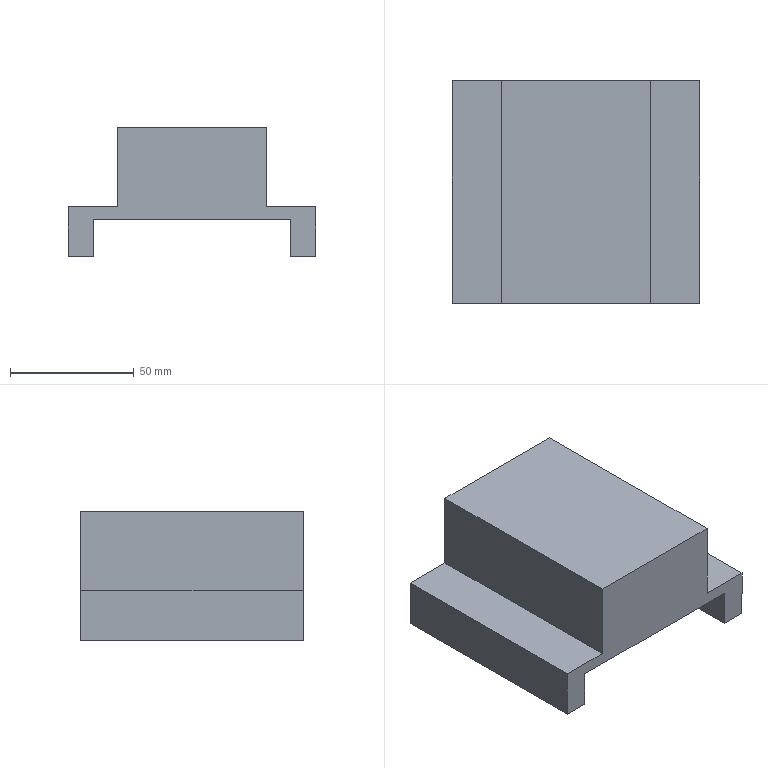Component | SolidWorks | Y-AxisAssembly-1_Y-AxisSlider-1 | 1 solid | 32 faces | box 100 x 90 x 52 mm | volume 243104 mm3 | plane 20 | cylinder 12 | commonest cylinder face diameters 6 x12
build123d program:
from build123d import *

# Parameters (mm, degrees)
BOSS_EXTRUDE1_DEPTH = 90
SKETCH2_R           = 3
CUT_EXTRUDE1_DEPTH  = 10


with BuildPart() as part:
    # Sketch1 → Boss-Extrude1 (new body)
    with BuildSketch(Plane.XY):
        Polygon((-50, 32.6), (-40, 32.6), (-40, 17.6), (40, 17.6), (40, 32.6), (50, 32.6), (50, 12.6), (30, 12.6), (30, -19.4), (-30, -19.4), (-30, 12.6), (-50, 12.6), align=None)
    extrude(amount=BOSS_EXTRUDE1_DEPTH)

    # Sketch2 → Cut-Extrude1 (cut)
    with BuildSketch(Plane(origin=(0, 32.6, 0), x_dir=(1, 0, 0), z_dir=(0, 1, 0))):
        with Locations(Location((-45, -10, 0), (0, 0, 270))):
            Circle(SKETCH2_R)
        with Locations(Location((45, -10, 0), (0, 0, 270))):
            Circle(SKETCH2_R)
        with Locations(Location((45, -45, 0), (0, 0, 270))):
            Circle(SKETCH2_R)
        with Locations(Location((45, -80, 0), (0, 0, 270))):
            Circle(SKETCH2_R)
        with Locations(Location((-45, -45, 0), (0, 0, 270))):
            Circle(SKETCH2_R)
        with Locations(Location((-45, -80, 0), (0, 0, 270))):
            Circle(SKETCH2_R)
    extrude(amount=-CUT_EXTRUDE1_DEPTH, mode=Mode.SUBTRACT)


solid = part.part

# Placed as in the assembly
solid = solid.moved(Location((-28.271, -116.882, -53.9), (-90, 0, 0)))
STEP:
#1=COLOUR_RGB('',0.7922,0.8196,0.9333);
#2=FILL_AREA_STYLE_COLOUR('',#1);
#3=FILL_AREA_STYLE('',(#2));
#4=SURFACE_STYLE_FILL_AREA(#3);
#5=SURFACE_SIDE_STYLE('',(#4));
#6=SURFACE_STYLE_USAGE(.BOTH.,#5);
#7=PRESENTATION_STYLE_ASSIGNMENT((#6));
#8=CARTESIAN_POINT('',(0.6586,-4.09,-3.012));
#9=VERTEX_POINT('',#8);
#10=CARTESIAN_POINT('',(0.6586,-4.326,-3.012));
#11=VERTEX_POINT('',#10);
#12=CARTESIAN_POINT('',(0.6586,-4.208,-3.012));
#13=DIRECTION('',(-0.,0.,-1.));
#14=DIRECTION('',(-0.,-1.,0.));
#15=AXIS2_PLACEMENT_3D('',#12,#13,#14);
#16=CIRCLE('',#15,0.1181);
#17=EDGE_CURVE('',#9,#11,#16,.T.);
#18=ORIENTED_EDGE('',*,*,#17,.F.);
#19=CARTESIAN_POINT('',(0.6586,-4.09,-3.406));
#20=VERTEX_POINT('',#19);
#21=CARTESIAN_POINT('',(0.6586,-4.09,-3.012));
#22=DIRECTION('',(-0.,0.,-1.));
#23=VECTOR('',#22,39.37);
#24=LINE('',#21,#23);
#25=EDGE_CURVE('',#9,#20,#24,.T.);
#26=ORIENTED_EDGE('',*,*,#25,.T.);
#27=CARTESIAN_POINT('',(0.6586,-4.326,-3.406));
#28=VERTEX_POINT('',#27);
#29=CARTESIAN_POINT('',(0.6586,-4.208,-3.406));
#30=DIRECTION('',(-0.,0.,-1.));
#31=DIRECTION('',(-0.,-1.,0.));
#32=AXIS2_PLACEMENT_3D('',#29,#30,#31);
#33=CIRCLE('',#32,0.1181);
#34=EDGE_CURVE('',#20,#28,#33,.T.);
#35=ORIENTED_EDGE('',*,*,#34,.T.);
#36=CARTESIAN_POINT('',(0.6586,-4.326,-3.012));
#37=DIRECTION('',(-0.,0.,-1.));
#38=VECTOR('',#37,39.37);
#39=LINE('',#36,#38);
#40=EDGE_CURVE('',#11,#28,#39,.T.);
#41=ORIENTED_EDGE('',*,*,#40,.F.);
#42=EDGE_LOOP('',(#18,#26,#35,#41));
#43=FACE_OUTER_BOUND('',#42,.T.);
#44=CARTESIAN_POINT('',(0.6586,-4.208,-3.012));
#45=DIRECTION('',(-0.,0.,-1.));
#46=DIRECTION('',(-0.,-1.,0.));
#47=AXIS2_PLACEMENT_3D('',#44,#45,#46);
#48=CYLINDRICAL_SURFACE('',#47,0.1181);
#49=ADVANCED_FACE('',(#43),#48,.F.);
#50=CARTESIAN_POINT('',(0.6586,-2.712,-3.012));
#51=VERTEX_POINT('',#50);
#52=CARTESIAN_POINT('',(0.6586,-2.948,-3.012));
#53=VERTEX_POINT('',#52);
#54=CARTESIAN_POINT('',(0.6586,-2.83,-3.012));
#55=DIRECTION('',(-0.,0.,-1.));
#56=DIRECTION('',(-0.,-1.,0.));
#57=AXIS2_PLACEMENT_3D('',#54,#55,#56);
#58=CIRCLE('',#57,0.1181);
#59=EDGE_CURVE('',#51,#53,#58,.T.);
#60=ORIENTED_EDGE('',*,*,#59,.F.);
#61=CARTESIAN_POINT('',(0.6586,-2.712,-3.406));
#62=VERTEX_POINT('',#61);
#63=CARTESIAN_POINT('',(0.6586,-2.712,-3.012));
#64=DIRECTION('',(-0.,0.,-1.));
#65=VECTOR('',#64,39.37);
#66=LINE('',#63,#65);
#67=EDGE_CURVE('',#51,#62,#66,.T.);
#68=ORIENTED_EDGE('',*,*,#67,.T.);
#69=CARTESIAN_POINT('',(0.6586,-2.948,-3.406));
#70=VERTEX_POINT('',#69);
#71=CARTESIAN_POINT('',(0.6586,-2.83,-3.406));
#72=DIRECTION('',(-0.,0.,-1.));
#73=DIRECTION('',(-0.,-1.,0.));
#74=AXIS2_PLACEMENT_3D('',#71,#72,#73);
#75=CIRCLE('',#74,0.1181);
#76=EDGE_CURVE('',#62,#70,#75,.T.);
#77=ORIENTED_EDGE('',*,*,#76,.T.);
#78=CARTESIAN_POINT('',(0.6586,-2.948,-3.012));
#79=DIRECTION('',(-0.,0.,-1.));
#80=VECTOR('',#79,39.37);
#81=LINE('',#78,#80);
#82=EDGE_CURVE('',#53,#70,#81,.T.);
#83=ORIENTED_EDGE('',*,*,#82,.F.);
#84=EDGE_LOOP('',(#60,#68,#77,#83));
#85=FACE_OUTER_BOUND('',#84,.T.);
#86=CARTESIAN_POINT('',(0.6586,-2.83,-3.012));
#87=DIRECTION('',(-0.,0.,-1.));
#88=DIRECTION('',(-0.,-1.,0.));
#89=AXIS2_PLACEMENT_3D('',#86,#87,#88);
#90=CYLINDRICAL_SURFACE('',#89,0.1181);
#91=ADVANCED_FACE('',(#85),#90,.F.);
#92=CARTESIAN_POINT('',(-2.885,-4.09,-3.012));
#93=VERTEX_POINT('',#92);
#94=CARTESIAN_POINT('',(-2.885,-4.326,-3.012));
#95=VERTEX_POINT('',#94);
#96=CARTESIAN_POINT('',(-2.885,-4.208,-3.012));
#97=DIRECTION('',(-0.,0.,-1.));
#98=DIRECTION('',(0.,-1.,0.));
#99=AXIS2_PLACEMENT_3D('',#96,#97,#98);
#100=CIRCLE('',#99,0.1181);
#101=EDGE_CURVE('',#93,#95,#100,.T.);
#102=ORIENTED_EDGE('',*,*,#101,.F.);
#103=CARTESIAN_POINT('',(-2.885,-4.09,-3.406));
#104=VERTEX_POINT('',#103);
#105=CARTESIAN_POINT('',(-2.885,-4.09,-3.012));
#106=DIRECTION('',(-0.,0.,-1.));
#107=VECTOR('',#106,39.37);
#108=LINE('',#105,#107);
#109=EDGE_CURVE('',#93,#104,#108,.T.);
#110=ORIENTED_EDGE('',*,*,#109,.T.);
#111=CARTESIAN_POINT('',(-2.885,-4.326,-3.406));
#112=VERTEX_POINT('',#111);
#113=CARTESIAN_POINT('',(-2.885,-4.208,-3.406));
#114=DIRECTION('',(-0.,0.,-1.));
#115=DIRECTION('',(0.,-1.,0.));
#116=AXIS2_PLACEMENT_3D('',#113,#114,#115);
#117=CIRCLE('',#116,0.1181);
#118=EDGE_CURVE('',#104,#112,#117,.T.);
#119=ORIENTED_EDGE('',*,*,#118,.T.);
#120=CARTESIAN_POINT('',(-2.885,-4.326,-3.012));
#121=DIRECTION('',(-0.,0.,-1.));
#122=VECTOR('',#121,39.37);
#123=LINE('',#120,#122);
#124=EDGE_CURVE('',#95,#112,#123,.T.);
#125=ORIENTED_EDGE('',*,*,#124,.F.);
#126=EDGE_LOOP('',(#102,#110,#119,#125));
#127=FACE_OUTER_BOUND('',#126,.T.);
#128=CARTESIAN_POINT('',(-2.885,-4.208,-3.012));
#129=DIRECTION('',(-0.,0.,-1.));
#130=DIRECTION('',(0.,-1.,0.));
#131=AXIS2_PLACEMENT_3D('',#128,#129,#130);
#132=CYLINDRICAL_SURFACE('',#131,0.1181);
#133=ADVANCED_FACE('',(#127),#132,.F.);
#134=CARTESIAN_POINT('',(-2.885,-2.712,-3.012));
#135=VERTEX_POINT('',#134);
#136=CARTESIAN_POINT('',(-2.885,-2.948,-3.012));
#137=VERTEX_POINT('',#136);
#138=CARTESIAN_POINT('',(-2.885,-2.83,-3.012));
#139=DIRECTION('',(-0.,0.,-1.));
#140=DIRECTION('',(0.,-1.,0.));
#141=AXIS2_PLACEMENT_3D('',#138,#139,#140);
#142=CIRCLE('',#141,0.1181);
#143=EDGE_CURVE('',#135,#137,#142,.T.);
#144=ORIENTED_EDGE('',*,*,#143,.F.);
#145=CARTESIAN_POINT('',(-2.885,-2.712,-3.406));
#146=VERTEX_POINT('',#145);
#147=CARTESIAN_POINT('',(-2.885,-2.712,-3.012));
#148=DIRECTION('',(-0.,0.,-1.));
#149=VECTOR('',#148,39.37);
#150=LINE('',#147,#149);
#151=EDGE_CURVE('',#135,#146,#150,.T.);
#152=ORIENTED_EDGE('',*,*,#151,.T.);
#153=CARTESIAN_POINT('',(-2.885,-2.948,-3.406));
#154=VERTEX_POINT('',#153);
#155=CARTESIAN_POINT('',(-2.885,-2.83,-3.406));
#156=DIRECTION('',(-0.,0.,-1.));
#157=DIRECTION('',(0.,-1.,0.));
#158=AXIS2_PLACEMENT_3D('',#155,#156,#157);
#159=CIRCLE('',#158,0.1181);
#160=EDGE_CURVE('',#146,#154,#159,.T.);
#161=ORIENTED_EDGE('',*,*,#160,.T.);
#162=CARTESIAN_POINT('',(-2.885,-2.948,-3.012));
#163=DIRECTION('',(-0.,0.,-1.));
#164=VECTOR('',#163,39.37);
#165=LINE('',#162,#164);
#166=EDGE_CURVE('',#137,#154,#165,.T.);
#167=ORIENTED_EDGE('',*,*,#166,.F.);
#168=EDGE_LOOP('',(#144,#152,#161,#167));
#169=FACE_OUTER_BOUND('',#168,.T.);
#170=CARTESIAN_POINT('',(-2.885,-2.83,-3.012));
#171=DIRECTION('',(-0.,0.,-1.));
#172=DIRECTION('',(0.,-1.,0.));
#173=AXIS2_PLACEMENT_3D('',#170,#171,#172);
#174=CYLINDRICAL_SURFACE('',#173,0.1181);
#175=ADVANCED_FACE('',(#169),#174,.F.);
#176=CARTESIAN_POINT('',(-2.885,-1.334,-3.012));
#177=VERTEX_POINT('',#176);
#178=CARTESIAN_POINT('',(-2.885,-1.57,-3.012));
#179=VERTEX_POINT('',#178);
#180=CARTESIAN_POINT('',(-2.885,-1.452,-3.012));
#181=DIRECTION('',(-0.,0.,-1.));
#182=DIRECTION('',(0.,-1.,0.));
#183=AXIS2_PLACEMENT_3D('',#180,#181,#182);
#184=CIRCLE('',#183,0.1181);
#185=EDGE_CURVE('',#177,#179,#184,.T.);
#186=ORIENTED_EDGE('',*,*,#185,.F.);
#187=CARTESIAN_POINT('',(-2.885,-1.334,-3.406));
#188=VERTEX_POINT('',#187);
#189=CARTESIAN_POINT('',(-2.885,-1.334,-3.012));
#190=DIRECTION('',(-0.,0.,-1.));
#191=VECTOR('',#190,39.37);
#192=LINE('',#189,#191);
#193=EDGE_CURVE('',#177,#188,#192,.T.);
#194=ORIENTED_EDGE('',*,*,#193,.T.);
#195=CARTESIAN_POINT('',(-2.885,-1.57,-3.406));
#196=VERTEX_POINT('',#195);
#197=CARTESIAN_POINT('',(-2.885,-1.452,-3.406));
#198=DIRECTION('',(-0.,0.,-1.));
#199=DIRECTION('',(0.,-1.,0.));
#200=AXIS2_PLACEMENT_3D('',#197,#198,#199);
#201=CIRCLE('',#200,0.1181);
#202=EDGE_CURVE('',#188,#196,#201,.T.);
#203=ORIENTED_EDGE('',*,*,#202,.T.);
#204=CARTESIAN_POINT('',(-2.885,-1.57,-3.012));
#205=DIRECTION('',(-0.,0.,-1.));
#206=VECTOR('',#205,39.37);
#207=LINE('',#204,#206);
#208=EDGE_CURVE('',#179,#196,#207,.T.);
#209=ORIENTED_EDGE('',*,*,#208,.F.);
#210=EDGE_LOOP('',(#186,#194,#203,#209));
#211=FACE_OUTER_BOUND('',#210,.T.);
#212=CARTESIAN_POINT('',(-2.885,-1.452,-3.012));
#213=DIRECTION('',(-0.,0.,-1.));
#214=DIRECTION('',(0.,-1.,0.));
#215=AXIS2_PLACEMENT_3D('',#212,#213,#214);
#216=CYLINDRICAL_SURFACE('',#215,0.1181);
#217=ADVANCED_FACE('',(#211),#216,.F.);
#218=CARTESIAN_POINT('',(0.6586,-1.334,-3.012));
#219=VERTEX_POINT('',#218);
#220=CARTESIAN_POINT('',(0.6586,-1.57,-3.012));
#221=VERTEX_POINT('',#220);
#222=CARTESIAN_POINT('',(0.6586,-1.452,-3.012));
#223=DIRECTION('',(-0.,0.,-1.));
#224=DIRECTION('',(-0.,-1.,0.));
#225=AXIS2_PLACEMENT_3D('',#222,#223,#224);
#226=CIRCLE('',#225,0.1181);
#227=EDGE_CURVE('',#219,#221,#226,.T.);
#228=ORIENTED_EDGE('',*,*,#227,.F.);
#229=CARTESIAN_POINT('',(0.6586,-1.334,-3.406));
#230=VERTEX_POINT('',#229);
#231=CARTESIAN_POINT('',(0.6586,-1.334,-3.012));
#232=DIRECTION('',(-0.,0.,-1.));
#233=VECTOR('',#232,39.37);
#234=LINE('',#231,#233);
#235=EDGE_CURVE('',#219,#230,#234,.T.);
#236=ORIENTED_EDGE('',*,*,#235,.T.);
#237=CARTESIAN_POINT('',(0.6586,-1.57,-3.406));
#238=VERTEX_POINT('',#237);
#239=CARTESIAN_POINT('',(0.6586,-1.452,-3.406));
#240=DIRECTION('',(-0.,0.,-1.));
#241=DIRECTION('',(-0.,-1.,0.));
#242=AXIS2_PLACEMENT_3D('',#239,#240,#241);
#243=CIRCLE('',#242,0.1181);
#244=EDGE_CURVE('',#230,#238,#243,.T.);
#245=ORIENTED_EDGE('',*,*,#244,.T.);
#246=CARTESIAN_POINT('',(0.6586,-1.57,-3.012));
#247=DIRECTION('',(-0.,0.,-1.));
#248=VECTOR('',#247,39.37);
#249=LINE('',#246,#248);
#250=EDGE_CURVE('',#221,#238,#249,.T.);
#251=ORIENTED_EDGE('',*,*,#250,.F.);
#252=EDGE_LOOP('',(#228,#236,#245,#251));
#253=FACE_OUTER_BOUND('',#252,.T.);
#254=CARTESIAN_POINT('',(0.6586,-1.452,-3.012));
#255=DIRECTION('',(-0.,0.,-1.));
#256=DIRECTION('',(-0.,-1.,0.));
#257=AXIS2_PLACEMENT_3D('',#254,#255,#256);
#258=CYLINDRICAL_SURFACE('',#257,0.1181);
#259=ADVANCED_FACE('',(#253),#258,.F.);
#260=CARTESIAN_POINT('',(0.8555,-1.058,-3.406));
#261=VERTEX_POINT('',#260);
#262=CARTESIAN_POINT('',(0.8555,-1.058,-2.618));
#263=VERTEX_POINT('',#262);
#264=CARTESIAN_POINT('',(0.8555,-1.058,-2.618));
#265=DIRECTION('',(0.,-0.,1.));
#266=VECTOR('',#265,39.37);
#267=LINE('',#264,#266);
#268=EDGE_CURVE('',#261,#263,#267,.T.);
#269=ORIENTED_EDGE('',*,*,#268,.T.);
#270=CARTESIAN_POINT('',(0.8555,-4.602,-2.618));
#271=VERTEX_POINT('',#270);
#272=CARTESIAN_POINT('',(0.8555,-4.602,-2.618));
#273=DIRECTION('',(0.,1.,0.));
#274=VECTOR('',#273,39.37);
#275=LINE('',#272,#274);
#276=EDGE_CURVE('',#271,#263,#275,.T.);
#277=ORIENTED_EDGE('',*,*,#276,.F.);
#278=CARTESIAN_POINT('',(0.8555,-4.602,-3.406));
#279=VERTEX_POINT('',#278);
#280=CARTESIAN_POINT('',(0.8555,-4.602,-2.618));
#281=DIRECTION('',(0.,-0.,1.));
#282=VECTOR('',#281,39.37);
#283=LINE('',#280,#282);
#284=EDGE_CURVE('',#279,#271,#283,.T.);
#285=ORIENTED_EDGE('',*,*,#284,.F.);
#286=CARTESIAN_POINT('',(0.8555,-4.602,-3.406));
#287=DIRECTION('',(0.,1.,0.));
#288=VECTOR('',#287,39.37);
#289=LINE('',#286,#288);
#290=EDGE_CURVE('',#279,#261,#289,.T.);
#291=ORIENTED_EDGE('',*,*,#290,.T.);
#292=EDGE_LOOP('',(#269,#277,#285,#291));
#293=FACE_OUTER_BOUND('',#292,.T.);
#294=CARTESIAN_POINT('',(0.8555,-4.602,-2.618));
#295=DIRECTION('',(-1.,0.,0.));
#296=DIRECTION('',(0.,1.,0.));
#297=AXIS2_PLACEMENT_3D('',#294,#295,#296);
#298=PLANE('',#297);
#299=ADVANCED_FACE('',(#293),#298,.F.);
#300=CARTESIAN_POINT('',(0.06809,-1.058,-2.618));
#301=VERTEX_POINT('',#300);
#302=CARTESIAN_POINT('',(0.06809,-1.058,-2.618));
#303=DIRECTION('',(-1.,0.,-0.));
#304=VECTOR('',#303,39.37);
#305=LINE('',#302,#304);
#306=EDGE_CURVE('',#263,#301,#305,.T.);
#307=ORIENTED_EDGE('',*,*,#306,.T.);
#308=CARTESIAN_POINT('',(0.06809,-4.602,-2.618));
#309=VERTEX_POINT('',#308);
#310=CARTESIAN_POINT('',(0.06809,-4.602,-2.618));
#311=DIRECTION('',(0.,1.,0.));
#312=VECTOR('',#311,39.37);
#313=LINE('',#310,#312);
#314=EDGE_CURVE('',#309,#301,#313,.T.);
#315=ORIENTED_EDGE('',*,*,#314,.F.);
#316=CARTESIAN_POINT('',(0.06809,-4.602,-2.618));
#317=DIRECTION('',(-1.,0.,-0.));
#318=VECTOR('',#317,39.37);
#319=LINE('',#316,#318);
#320=EDGE_CURVE('',#271,#309,#319,.T.);
#321=ORIENTED_EDGE('',*,*,#320,.F.);
#322=ORIENTED_EDGE('',*,*,#276,.T.);
#323=EDGE_LOOP('',(#307,#315,#321,#322));
#324=FACE_OUTER_BOUND('',#323,.T.);
#325=CARTESIAN_POINT('',(0.06809,-4.602,-2.618));
#326=DIRECTION('',(0.,0.,-1.));
#327=DIRECTION('',(1.,-0.,0.));
#328=AXIS2_PLACEMENT_3D('',#325,#326,#327);
#329=PLANE('',#328);
#330=ADVANCED_FACE('',(#324),#329,.F.);
#331=CARTESIAN_POINT('',(0.06809,-1.058,-1.358));
#332=VERTEX_POINT('',#331);
#333=CARTESIAN_POINT('',(0.06809,-1.058,-1.358));
#334=DIRECTION('',(0.,-0.,1.));
#335=VECTOR('',#334,39.37);
#336=LINE('',#333,#335);
#337=EDGE_CURVE('',#301,#332,#336,.T.);
#338=ORIENTED_EDGE('',*,*,#337,.T.);
#339=CARTESIAN_POINT('',(0.06809,-4.602,-1.358));
#340=VERTEX_POINT('',#339);
#341=CARTESIAN_POINT('',(0.06809,-4.602,-1.358));
#342=DIRECTION('',(0.,1.,0.));
#343=VECTOR('',#342,39.37);
#344=LINE('',#341,#343);
#345=EDGE_CURVE('',#340,#332,#344,.T.);
#346=ORIENTED_EDGE('',*,*,#345,.F.);
#347=CARTESIAN_POINT('',(0.06809,-4.602,-1.358));
#348=DIRECTION('',(0.,-0.,1.));
#349=VECTOR('',#348,39.37);
#350=LINE('',#347,#349);
#351=EDGE_CURVE('',#309,#340,#350,.T.);
#352=ORIENTED_EDGE('',*,*,#351,.F.);
#353=ORIENTED_EDGE('',*,*,#314,.T.);
#354=EDGE_LOOP('',(#338,#346,#352,#353));
#355=FACE_OUTER_BOUND('',#354,.T.);
#356=CARTESIAN_POINT('',(0.06809,-4.602,-1.358));
#357=DIRECTION('',(-1.,0.,0.));
#358=DIRECTION('',(0.,1.,0.));
#359=AXIS2_PLACEMENT_3D('',#356,#357,#358);
#360=PLANE('',#359);
#361=ADVANCED_FACE('',(#355),#360,.F.);
#362=CARTESIAN_POINT('',(-2.294,-1.058,-1.358));
#363=VERTEX_POINT('',#362);
#364=CARTESIAN_POINT('',(-2.294,-1.058,-1.358));
#365=DIRECTION('',(-1.,0.,0.));
#366=VECTOR('',#365,39.37);
#367=LINE('',#364,#366);
#368=EDGE_CURVE('',#332,#363,#367,.T.);
#369=ORIENTED_EDGE('',*,*,#368,.T.);
#370=CARTESIAN_POINT('',(-2.294,-4.602,-1.358));
#371=VERTEX_POINT('',#370);
#372=CARTESIAN_POINT('',(-2.294,-4.602,-1.358));
#373=DIRECTION('',(0.,1.,0.));
#374=VECTOR('',#373,39.37);
#375=LINE('',#372,#374);
#376=EDGE_CURVE('',#371,#363,#375,.T.);
#377=ORIENTED_EDGE('',*,*,#376,.F.);
#378=CARTESIAN_POINT('',(-2.294,-4.602,-1.358));
#379=DIRECTION('',(-1.,0.,0.));
#380=VECTOR('',#379,39.37);
#381=LINE('',#378,#380);
#382=EDGE_CURVE('',#340,#371,#381,.T.);
#383=ORIENTED_EDGE('',*,*,#382,.F.);
#384=ORIENTED_EDGE('',*,*,#345,.T.);
#385=EDGE_LOOP('',(#369,#377,#383,#384));
#386=FACE_OUTER_BOUND('',#385,.T.);
#387=CARTESIAN_POINT('',(-2.294,-4.602,-1.358));
#388=DIRECTION('',(-0.,0.,-1.));
#389=DIRECTION('',(1.,-0.,-0.));
#390=AXIS2_PLACEMENT_3D('',#387,#388,#389);
#391=PLANE('',#390);
#392=ADVANCED_FACE('',(#386),#391,.F.);
#393=CARTESIAN_POINT('',(-2.294,-1.058,-2.618));
#394=VERTEX_POINT('',#393);
#395=CARTESIAN_POINT('',(-2.294,-1.058,-2.618));
#396=DIRECTION('',(0.,0.,-1.));
#397=VECTOR('',#396,39.37);
#398=LINE('',#395,#397);
#399=EDGE_CURVE('',#363,#394,#398,.T.);
#400=ORIENTED_EDGE('',*,*,#399,.T.);
#401=CARTESIAN_POINT('',(-2.294,-4.602,-2.618));
#402=VERTEX_POINT('',#401);
#403=CARTESIAN_POINT('',(-2.294,-4.602,-2.618));
#404=DIRECTION('',(0.,1.,0.));
#405=VECTOR('',#404,39.37);
#406=LINE('',#403,#405);
#407=EDGE_CURVE('',#402,#394,#406,.T.);
#408=ORIENTED_EDGE('',*,*,#407,.F.);
#409=CARTESIAN_POINT('',(-2.294,-4.602,-2.618));
#410=DIRECTION('',(0.,0.,-1.));
#411=VECTOR('',#410,39.37);
#412=LINE('',#409,#411);
#413=EDGE_CURVE('',#371,#402,#412,.T.);
#414=ORIENTED_EDGE('',*,*,#413,.F.);
#415=ORIENTED_EDGE('',*,*,#376,.T.);
#416=EDGE_LOOP('',(#400,#408,#414,#415));
#417=FACE_OUTER_BOUND('',#416,.T.);
#418=CARTESIAN_POINT('',(-2.294,-4.602,-2.618));
#419=DIRECTION('',(1.,-0.,0.));
#420=DIRECTION('',(-0.,-0.,1.));
#421=AXIS2_PLACEMENT_3D('',#418,#419,#420);
#422=PLANE('',#421);
#423=ADVANCED_FACE('',(#417),#422,.F.);
#424=CARTESIAN_POINT('',(-3.082,-1.058,-2.618));
#425=VERTEX_POINT('',#424);
#426=CARTESIAN_POINT('',(-3.082,-1.058,-2.618));
#427=DIRECTION('',(-1.,0.,0.));
#428=VECTOR('',#427,39.37);
#429=LINE('',#426,#428);
#430=EDGE_CURVE('',#394,#425,#429,.T.);
#431=ORIENTED_EDGE('',*,*,#430,.T.);
#432=CARTESIAN_POINT('',(-3.082,-4.602,-2.618));
#433=VERTEX_POINT('',#432);
#434=CARTESIAN_POINT('',(-3.082,-4.602,-2.618));
#435=DIRECTION('',(0.,1.,0.));
#436=VECTOR('',#435,39.37);
#437=LINE('',#434,#436);
#438=EDGE_CURVE('',#433,#425,#437,.T.);
#439=ORIENTED_EDGE('',*,*,#438,.F.);
#440=CARTESIAN_POINT('',(-3.082,-4.602,-2.618));
#441=DIRECTION('',(-1.,0.,0.));
#442=VECTOR('',#441,39.37);
#443=LINE('',#440,#442);
#444=EDGE_CURVE('',#402,#433,#443,.T.);
#445=ORIENTED_EDGE('',*,*,#444,.F.);
#446=ORIENTED_EDGE('',*,*,#407,.T.);
#447=EDGE_LOOP('',(#431,#439,#445,#446));
#448=FACE_OUTER_BOUND('',#447,.T.);
#449=CARTESIAN_POINT('',(-3.082,-4.602,-2.618));
#450=DIRECTION('',(-0.,0.,-1.));
#451=DIRECTION('',(1.,-0.,-0.));
#452=AXIS2_PLACEMENT_3D('',#449,#450,#451);
#453=PLANE('',#452);
#454=ADVANCED_FACE('',(#448),#453,.F.);
#455=CARTESIAN_POINT('',(-3.082,-1.058,-3.406));
#456=VERTEX_POINT('',#455);
#457=CARTESIAN_POINT('',(-3.082,-1.058,-3.406));
#458=DIRECTION('',(-0.,0.,-1.));
#459=VECTOR('',#458,39.37);
#460=LINE('',#457,#459);
#461=EDGE_CURVE('',#425,#456,#460,.T.);
#462=ORIENTED_EDGE('',*,*,#461,.T.);
#463=CARTESIAN_POINT('',(-3.082,-4.602,-3.406));
#464=VERTEX_POINT('',#463);
#465=CARTESIAN_POINT('',(-3.082,-4.602,-3.406));
#466=DIRECTION('',(0.,1.,0.));
#467=VECTOR('',#466,39.37);
#468=LINE('',#465,#467);
#469=EDGE_CURVE('',#464,#456,#468,.T.);
#470=ORIENTED_EDGE('',*,*,#469,.F.);
#471=CARTESIAN_POINT('',(-3.082,-4.602,-3.406));
#472=DIRECTION('',(-0.,0.,-1.));
#473=VECTOR('',#472,39.37);
#474=LINE('',#471,#473);
#475=EDGE_CURVE('',#433,#464,#474,.T.);
#476=ORIENTED_EDGE('',*,*,#475,.F.);
#477=ORIENTED_EDGE('',*,*,#438,.T.);
#478=EDGE_LOOP('',(#462,#470,#476,#477));
#479=FACE_OUTER_BOUND('',#478,.T.);
#480=CARTESIAN_POINT('',(-3.082,-4.602,-3.406));
#481=DIRECTION('',(1.,-0.,-0.));
#482=DIRECTION('',(-0.,-1.,-0.));
#483=AXIS2_PLACEMENT_3D('',#480,#481,#482);
#484=PLANE('',#483);
#485=ADVANCED_FACE('',(#479),#484,.F.);
#486=CARTESIAN_POINT('',(-2.885,-4.208,-3.406));
#487=DIRECTION('',(-0.,0.,-1.));
#488=DIRECTION('',(0.,-1.,0.));
#489=AXIS2_PLACEMENT_3D('',#486,#487,#488);
#490=CIRCLE('',#489,0.1181);
#491=EDGE_CURVE('',#112,#104,#490,.T.);
#492=ORIENTED_EDGE('',*,*,#491,.F.);
#493=ORIENTED_EDGE('',*,*,#118,.F.);
#494=EDGE_LOOP('',(#492,#493));
#495=FACE_BOUND('',#494,.T.);
#496=CARTESIAN_POINT('',(-2.885,-2.83,-3.406));
#497=DIRECTION('',(-0.,0.,-1.));
#498=DIRECTION('',(0.,-1.,0.));
#499=AXIS2_PLACEMENT_3D('',#496,#497,#498);
#500=CIRCLE('',#499,0.1181);
#501=EDGE_CURVE('',#154,#146,#500,.T.);
#502=ORIENTED_EDGE('',*,*,#501,.F.);
#503=ORIENTED_EDGE('',*,*,#160,.F.);
#504=EDGE_LOOP('',(#502,#503));
#505=FACE_BOUND('',#504,.T.);
#506=CARTESIAN_POINT('',(-2.885,-1.452,-3.406));
#507=DIRECTION('',(-0.,0.,-1.));
#508=DIRECTION('',(0.,-1.,0.));
#509=AXIS2_PLACEMENT_3D('',#506,#507,#508);
#510=CIRCLE('',#509,0.1181);
#511=EDGE_CURVE('',#196,#188,#510,.T.);
#512=ORIENTED_EDGE('',*,*,#511,.F.);
#513=ORIENTED_EDGE('',*,*,#202,.F.);
#514=EDGE_LOOP('',(#512,#513));
#515=FACE_BOUND('',#514,.T.);
#516=CARTESIAN_POINT('',(-2.688,-1.058,-3.406));
#517=VERTEX_POINT('',#516);
#518=CARTESIAN_POINT('',(-2.688,-1.058,-3.406));
#519=DIRECTION('',(1.,-0.,-0.));
#520=VECTOR('',#519,39.37);
#521=LINE('',#518,#520);
#522=EDGE_CURVE('',#456,#517,#521,.T.);
#523=ORIENTED_EDGE('',*,*,#522,.T.);
#524=CARTESIAN_POINT('',(-2.688,-4.602,-3.406));
#525=VERTEX_POINT('',#524);
#526=CARTESIAN_POINT('',(-2.688,-4.602,-3.406));
#527=DIRECTION('',(0.,1.,0.));
#528=VECTOR('',#527,39.37);
#529=LINE('',#526,#528);
#530=EDGE_CURVE('',#525,#517,#529,.T.);
#531=ORIENTED_EDGE('',*,*,#530,.F.);
#532=CARTESIAN_POINT('',(-2.688,-4.602,-3.406));
#533=DIRECTION('',(1.,-0.,-0.));
#534=VECTOR('',#533,39.37);
#535=LINE('',#532,#534);
#536=EDGE_CURVE('',#464,#525,#535,.T.);
#537=ORIENTED_EDGE('',*,*,#536,.F.);
#538=ORIENTED_EDGE('',*,*,#469,.T.);
#539=EDGE_LOOP('',(#523,#531,#537,#538));
#540=FACE_OUTER_BOUND('',#539,.T.);
#541=CARTESIAN_POINT('',(-2.688,-4.602,-3.406));
#542=DIRECTION('',(0.,-0.,1.));
#543=DIRECTION('',(0.,1.,0.));
#544=AXIS2_PLACEMENT_3D('',#541,#542,#543);
#545=PLANE('',#544);
#546=ADVANCED_FACE('',(#495,#505,#515,#540),#545,.F.);
#547=CARTESIAN_POINT('',(-2.688,-1.058,-2.815));
#548=VERTEX_POINT('',#547);
#549=CARTESIAN_POINT('',(-2.688,-1.058,-2.815));
#550=DIRECTION('',(0.,-0.,1.));
#551=VECTOR('',#550,39.37);
#552=LINE('',#549,#551);
#553=EDGE_CURVE('',#517,#548,#552,.T.);
#554=ORIENTED_EDGE('',*,*,#553,.T.);
#555=CARTESIAN_POINT('',(-2.688,-4.602,-2.815));
#556=VERTEX_POINT('',#555);
#557=CARTESIAN_POINT('',(-2.688,-4.602,-2.815));
#558=DIRECTION('',(0.,1.,0.));
#559=VECTOR('',#558,39.37);
#560=LINE('',#557,#559);
#561=EDGE_CURVE('',#556,#548,#560,.T.);
#562=ORIENTED_EDGE('',*,*,#561,.F.);
#563=CARTESIAN_POINT('',(-2.688,-4.602,-2.815));
#564=DIRECTION('',(0.,-0.,1.));
#565=VECTOR('',#564,39.37);
#566=LINE('',#563,#565);
#567=EDGE_CURVE('',#525,#556,#566,.T.);
#568=ORIENTED_EDGE('',*,*,#567,.F.);
#569=ORIENTED_EDGE('',*,*,#530,.T.);
#570=EDGE_LOOP('',(#554,#562,#568,#569));
#571=FACE_OUTER_BOUND('',#570,.T.);
#572=CARTESIAN_POINT('',(-2.688,-4.602,-2.815));
#573=DIRECTION('',(-1.,0.,0.));
#574=DIRECTION('',(0.,1.,0.));
#575=AXIS2_PLACEMENT_3D('',#572,#573,#574);
#576=PLANE('',#575);
#577=ADVANCED_FACE('',(#571),#576,.F.);
#578=CARTESIAN_POINT('',(0.4618,-1.058,-2.815));
#579=VERTEX_POINT('',#578);
#580=CARTESIAN_POINT('',(0.4618,-1.058,-2.815));
#581=DIRECTION('',(1.,-0.,-0.));
#582=VECTOR('',#581,39.37);
#583=LINE('',#580,#582);
#584=EDGE_CURVE('',#548,#579,#583,.T.);
#585=ORIENTED_EDGE('',*,*,#584,.T.);
#586=CARTESIAN_POINT('',(0.4618,-4.602,-2.815));
#587=VERTEX_POINT('',#586);
#588=CARTESIAN_POINT('',(0.4618,-4.602,-2.815));
#589=DIRECTION('',(0.,1.,0.));
#590=VECTOR('',#589,39.37);
#591=LINE('',#588,#590);
#592=EDGE_CURVE('',#587,#579,#591,.T.);
#593=ORIENTED_EDGE('',*,*,#592,.F.);
#594=CARTESIAN_POINT('',(0.4618,-4.602,-2.815));
#595=DIRECTION('',(1.,-0.,-0.));
#596=VECTOR('',#595,39.37);
#597=LINE('',#594,#596);
#598=EDGE_CURVE('',#556,#587,#597,.T.);
#599=ORIENTED_EDGE('',*,*,#598,.F.);
#600=ORIENTED_EDGE('',*,*,#561,.T.);
#601=EDGE_LOOP('',(#585,#593,#599,#600));
#602=FACE_OUTER_BOUND('',#601,.T.);
#603=CARTESIAN_POINT('',(0.4618,-4.602,-2.815));
#604=DIRECTION('',(0.,-0.,1.));
#605=DIRECTION('',(0.,1.,0.));
#606=AXIS2_PLACEMENT_3D('',#603,#604,#605);
#607=PLANE('',#606);
#608=ADVANCED_FACE('',(#602),#607,.F.);
#609=CARTESIAN_POINT('',(0.4618,-1.058,-3.406));
#610=VERTEX_POINT('',#609);
#611=CARTESIAN_POINT('',(0.4618,-1.058,-3.406));
#612=DIRECTION('',(-0.,0.,-1.));
#613=VECTOR('',#612,39.37);
#614=LINE('',#611,#613);
#615=EDGE_CURVE('',#579,#610,#614,.T.);
#616=ORIENTED_EDGE('',*,*,#615,.T.);
#617=CARTESIAN_POINT('',(0.4618,-4.602,-3.406));
#618=VERTEX_POINT('',#617);
#619=CARTESIAN_POINT('',(0.4618,-4.602,-3.406));
#620=DIRECTION('',(0.,1.,0.));
#621=VECTOR('',#620,39.37);
#622=LINE('',#619,#621);
#623=EDGE_CURVE('',#618,#610,#622,.T.);
#624=ORIENTED_EDGE('',*,*,#623,.F.);
#625=CARTESIAN_POINT('',(0.4618,-4.602,-3.406));
#626=DIRECTION('',(-0.,0.,-1.));
#627=VECTOR('',#626,39.37);
#628=LINE('',#625,#627);
#629=EDGE_CURVE('',#587,#618,#628,.T.);
#630=ORIENTED_EDGE('',*,*,#629,.F.);
#631=ORIENTED_EDGE('',*,*,#592,.T.);
#632=EDGE_LOOP('',(#616,#624,#630,#631));
#633=FACE_OUTER_BOUND('',#632,.T.);
#634=CARTESIAN_POINT('',(0.4618,-4.602,-3.406));
#635=DIRECTION('',(1.,-0.,-0.));
#636=DIRECTION('',(-0.,-1.,-0.));
#637=AXIS2_PLACEMENT_3D('',#634,#635,#636);
#638=PLANE('',#637);
#639=ADVANCED_FACE('',(#633),#638,.F.);
#640=CARTESIAN_POINT('',(0.6586,-4.208,-3.406));
#641=DIRECTION('',(-0.,0.,-1.));
#642=DIRECTION('',(-0.,-1.,0.));
#643=AXIS2_PLACEMENT_3D('',#640,#641,#642);
#644=CIRCLE('',#643,0.1181);
#645=EDGE_CURVE('',#28,#20,#644,.T.);
#646=ORIENTED_EDGE('',*,*,#645,.F.);
#647=ORIENTED_EDGE('',*,*,#34,.F.);
#648=EDGE_LOOP('',(#646,#647));
#649=FACE_BOUND('',#648,.T.);
#650=CARTESIAN_POINT('',(0.6586,-2.83,-3.406));
#651=DIRECTION('',(-0.,0.,-1.));
#652=DIRECTION('',(-0.,-1.,0.));
#653=AXIS2_PLACEMENT_3D('',#650,#651,#652);
#654=CIRCLE('',#653,0.1181);
#655=EDGE_CURVE('',#70,#62,#654,.T.);
#656=ORIENTED_EDGE('',*,*,#655,.F.);
#657=ORIENTED_EDGE('',*,*,#76,.F.);
#658=EDGE_LOOP('',(#656,#657));
#659=FACE_BOUND('',#658,.T.);
#660=CARTESIAN_POINT('',(0.6586,-1.452,-3.406));
#661=DIRECTION('',(-0.,0.,-1.));
#662=DIRECTION('',(-0.,-1.,0.));
#663=AXIS2_PLACEMENT_3D('',#660,#661,#662);
#664=CIRCLE('',#663,0.1181);
#665=EDGE_CURVE('',#238,#230,#664,.T.);
#666=ORIENTED_EDGE('',*,*,#665,.F.);
#667=ORIENTED_EDGE('',*,*,#244,.F.);
#668=EDGE_LOOP('',(#666,#667));
#669=FACE_BOUND('',#668,.T.);
#670=CARTESIAN_POINT('',(0.8555,-1.058,-3.406));
#671=DIRECTION('',(1.,-0.,-0.));
#672=VECTOR('',#671,39.37);
#673=LINE('',#670,#672);
#674=EDGE_CURVE('',#610,#261,#673,.T.);
#675=ORIENTED_EDGE('',*,*,#674,.T.);
#676=ORIENTED_EDGE('',*,*,#290,.F.);
#677=CARTESIAN_POINT('',(0.8555,-4.602,-3.406));
#678=DIRECTION('',(1.,-0.,-0.));
#679=VECTOR('',#678,39.37);
#680=LINE('',#677,#679);
#681=EDGE_CURVE('',#618,#279,#680,.T.);
#682=ORIENTED_EDGE('',*,*,#681,.F.);
#683=ORIENTED_EDGE('',*,*,#623,.T.);
#684=EDGE_LOOP('',(#675,#676,#682,#683));
#685=FACE_OUTER_BOUND('',#684,.T.);
#686=CARTESIAN_POINT('',(0.8555,-4.602,-3.406));
#687=DIRECTION('',(0.,-0.,1.));
#688=DIRECTION('',(0.,1.,0.));
#689=AXIS2_PLACEMENT_3D('',#686,#687,#688);
#690=PLANE('',#689);
#691=ADVANCED_FACE('',(#649,#659,#669,#685),#690,.F.);
#692=ORIENTED_EDGE('',*,*,#284,.T.);
#693=ORIENTED_EDGE('',*,*,#320,.T.);
#694=ORIENTED_EDGE('',*,*,#351,.T.);
#695=ORIENTED_EDGE('',*,*,#382,.T.);
#696=ORIENTED_EDGE('',*,*,#413,.T.);
#697=ORIENTED_EDGE('',*,*,#444,.T.);
#698=ORIENTED_EDGE('',*,*,#475,.T.);
#699=ORIENTED_EDGE('',*,*,#536,.T.);
#700=ORIENTED_EDGE('',*,*,#567,.T.);
#701=ORIENTED_EDGE('',*,*,#598,.T.);
#702=ORIENTED_EDGE('',*,*,#629,.T.);
#703=ORIENTED_EDGE('',*,*,#681,.T.);
#704=EDGE_LOOP('',(#692,#693,#694,#695,#696,#697,#698,#699,#700,#701,#702,#703));
#705=FACE_OUTER_BOUND('',#704,.T.);
#706=CARTESIAN_POINT('',(-1.113,-4.602,-2.122));
#707=DIRECTION('',(0.,1.,0.));
#708=DIRECTION('',(1.,-0.,-0.));
#709=AXIS2_PLACEMENT_3D('',#706,#707,#708);
#710=PLANE('',#709);
#711=ADVANCED_FACE('',(#705),#710,.F.);
#712=ORIENTED_EDGE('',*,*,#268,.F.);
#713=ORIENTED_EDGE('',*,*,#674,.F.);
#714=ORIENTED_EDGE('',*,*,#615,.F.);
#715=ORIENTED_EDGE('',*,*,#584,.F.);
#716=ORIENTED_EDGE('',*,*,#553,.F.);
#717=ORIENTED_EDGE('',*,*,#522,.F.);
#718=ORIENTED_EDGE('',*,*,#461,.F.);
#719=ORIENTED_EDGE('',*,*,#430,.F.);
#720=ORIENTED_EDGE('',*,*,#399,.F.);
#721=ORIENTED_EDGE('',*,*,#368,.F.);
#722=ORIENTED_EDGE('',*,*,#337,.F.);
#723=ORIENTED_EDGE('',*,*,#306,.F.);
#724=EDGE_LOOP('',(#712,#713,#714,#715,#716,#717,#718,#719,#720,#721,#722,#723));
#725=FACE_OUTER_BOUND('',#724,.T.);
#726=CARTESIAN_POINT('',(-1.113,-1.058,-2.122));
#727=DIRECTION('',(0.,1.,0.));
#728=DIRECTION('',(1.,-0.,-0.));
#729=AXIS2_PLACEMENT_3D('',#726,#727,#728);
#730=PLANE('',#729);
#731=ADVANCED_FACE('',(#725),#730,.T.);
#732=ORIENTED_EDGE('',*,*,#235,.F.);
#733=CARTESIAN_POINT('',(0.6586,-1.452,-3.012));
#734=DIRECTION('',(-0.,0.,-1.));
#735=DIRECTION('',(-0.,-1.,0.));
#736=AXIS2_PLACEMENT_3D('',#733,#734,#735);
#737=CIRCLE('',#736,0.1181);
#738=EDGE_CURVE('',#221,#219,#737,.T.);
#739=ORIENTED_EDGE('',*,*,#738,.F.);
#740=ORIENTED_EDGE('',*,*,#250,.T.);
#741=ORIENTED_EDGE('',*,*,#665,.T.);
#742=EDGE_LOOP('',(#732,#739,#740,#741));
#743=FACE_OUTER_BOUND('',#742,.T.);
#744=CARTESIAN_POINT('',(0.6586,-1.452,-3.012));
#745=DIRECTION('',(-0.,0.,-1.));
#746=DIRECTION('',(-0.,-1.,0.));
#747=AXIS2_PLACEMENT_3D('',#744,#745,#746);
#748=CYLINDRICAL_SURFACE('',#747,0.1181);
#749=ADVANCED_FACE('',(#743),#748,.F.);
#750=ORIENTED_EDGE('',*,*,#738,.T.);
#751=ORIENTED_EDGE('',*,*,#227,.T.);
#752=EDGE_LOOP('',(#750,#751));
#753=FACE_OUTER_BOUND('',#752,.T.);
#754=CARTESIAN_POINT('',(0.6586,-1.452,-3.012));
#755=DIRECTION('',(-0.,0.,-1.));
#756=DIRECTION('',(-0.,-1.,-0.));
#757=AXIS2_PLACEMENT_3D('',#754,#755,#756);
#758=PLANE('',#757);
#759=ADVANCED_FACE('',(#753),#758,.T.);
#760=ORIENTED_EDGE('',*,*,#193,.F.);
#761=CARTESIAN_POINT('',(-2.885,-1.452,-3.012));
#762=DIRECTION('',(-0.,0.,-1.));
#763=DIRECTION('',(0.,-1.,0.));
#764=AXIS2_PLACEMENT_3D('',#761,#762,#763);
#765=CIRCLE('',#764,0.1181);
#766=EDGE_CURVE('',#179,#177,#765,.T.);
#767=ORIENTED_EDGE('',*,*,#766,.F.);
#768=ORIENTED_EDGE('',*,*,#208,.T.);
#769=ORIENTED_EDGE('',*,*,#511,.T.);
#770=EDGE_LOOP('',(#760,#767,#768,#769));
#771=FACE_OUTER_BOUND('',#770,.T.);
#772=CARTESIAN_POINT('',(-2.885,-1.452,-3.012));
#773=DIRECTION('',(-0.,0.,-1.));
#774=DIRECTION('',(0.,-1.,0.));
#775=AXIS2_PLACEMENT_3D('',#772,#773,#774);
#776=CYLINDRICAL_SURFACE('',#775,0.1181);
#777=ADVANCED_FACE('',(#771),#776,.F.);
#778=ORIENTED_EDGE('',*,*,#766,.T.);
#779=ORIENTED_EDGE('',*,*,#185,.T.);
#780=EDGE_LOOP('',(#778,#779));
#781=FACE_OUTER_BOUND('',#780,.T.);
#782=CARTESIAN_POINT('',(-2.885,-1.452,-3.012));
#783=DIRECTION('',(-0.,0.,-1.));
#784=DIRECTION('',(-0.,-1.,-0.));
#785=AXIS2_PLACEMENT_3D('',#782,#783,#784);
#786=PLANE('',#785);
#787=ADVANCED_FACE('',(#781),#786,.T.);
#788=ORIENTED_EDGE('',*,*,#151,.F.);
#789=CARTESIAN_POINT('',(-2.885,-2.83,-3.012));
#790=DIRECTION('',(-0.,0.,-1.));
#791=DIRECTION('',(0.,-1.,0.));
#792=AXIS2_PLACEMENT_3D('',#789,#790,#791);
#793=CIRCLE('',#792,0.1181);
#794=EDGE_CURVE('',#137,#135,#793,.T.);
#795=ORIENTED_EDGE('',*,*,#794,.F.);
#796=ORIENTED_EDGE('',*,*,#166,.T.);
#797=ORIENTED_EDGE('',*,*,#501,.T.);
#798=EDGE_LOOP('',(#788,#795,#796,#797));
#799=FACE_OUTER_BOUND('',#798,.T.);
#800=CARTESIAN_POINT('',(-2.885,-2.83,-3.012));
#801=DIRECTION('',(-0.,0.,-1.));
#802=DIRECTION('',(0.,-1.,0.));
#803=AXIS2_PLACEMENT_3D('',#800,#801,#802);
#804=CYLINDRICAL_SURFACE('',#803,0.1181);
#805=ADVANCED_FACE('',(#799),#804,.F.);
#806=ORIENTED_EDGE('',*,*,#794,.T.);
#807=ORIENTED_EDGE('',*,*,#143,.T.);
#808=EDGE_LOOP('',(#806,#807));
#809=FACE_OUTER_BOUND('',#808,.T.);
#810=CARTESIAN_POINT('',(-2.885,-2.83,-3.012));
#811=DIRECTION('',(-0.,0.,-1.));
#812=DIRECTION('',(-0.,-1.,-0.));
#813=AXIS2_PLACEMENT_3D('',#810,#811,#812);
#814=PLANE('',#813);
#815=ADVANCED_FACE('',(#809),#814,.T.);
#816=ORIENTED_EDGE('',*,*,#109,.F.);
#817=CARTESIAN_POINT('',(-2.885,-4.208,-3.012));
#818=DIRECTION('',(-0.,0.,-1.));
#819=DIRECTION('',(0.,-1.,0.));
#820=AXIS2_PLACEMENT_3D('',#817,#818,#819);
#821=CIRCLE('',#820,0.1181);
#822=EDGE_CURVE('',#95,#93,#821,.T.);
#823=ORIENTED_EDGE('',*,*,#822,.F.);
#824=ORIENTED_EDGE('',*,*,#124,.T.);
#825=ORIENTED_EDGE('',*,*,#491,.T.);
#826=EDGE_LOOP('',(#816,#823,#824,#825));
#827=FACE_OUTER_BOUND('',#826,.T.);
#828=CARTESIAN_POINT('',(-2.885,-4.208,-3.012));
#829=DIRECTION('',(-0.,0.,-1.));
#830=DIRECTION('',(0.,-1.,0.));
#831=AXIS2_PLACEMENT_3D('',#828,#829,#830);
#832=CYLINDRICAL_SURFACE('',#831,0.1181);
#833=ADVANCED_FACE('',(#827),#832,.F.);
#834=ORIENTED_EDGE('',*,*,#822,.T.);
#835=ORIENTED_EDGE('',*,*,#101,.T.);
#836=EDGE_LOOP('',(#834,#835));
#837=FACE_OUTER_BOUND('',#836,.T.);
#838=CARTESIAN_POINT('',(-2.885,-4.208,-3.012));
#839=DIRECTION('',(-0.,0.,-1.));
#840=DIRECTION('',(-0.,-1.,-0.));
#841=AXIS2_PLACEMENT_3D('',#838,#839,#840);
#842=PLANE('',#841);
#843=ADVANCED_FACE('',(#837),#842,.T.);
#844=ORIENTED_EDGE('',*,*,#67,.F.);
#845=CARTESIAN_POINT('',(0.6586,-2.83,-3.012));
#846=DIRECTION('',(-0.,0.,-1.));
#847=DIRECTION('',(-0.,-1.,0.));
#848=AXIS2_PLACEMENT_3D('',#845,#846,#847);
#849=CIRCLE('',#848,0.1181);
#850=EDGE_CURVE('',#53,#51,#849,.T.);
#851=ORIENTED_EDGE('',*,*,#850,.F.);
#852=ORIENTED_EDGE('',*,*,#82,.T.);
#853=ORIENTED_EDGE('',*,*,#655,.T.);
#854=EDGE_LOOP('',(#844,#851,#852,#853));
#855=FACE_OUTER_BOUND('',#854,.T.);
#856=CARTESIAN_POINT('',(0.6586,-2.83,-3.012));
#857=DIRECTION('',(-0.,0.,-1.));
#858=DIRECTION('',(-0.,-1.,0.));
#859=AXIS2_PLACEMENT_3D('',#856,#857,#858);
#860=CYLINDRICAL_SURFACE('',#859,0.1181);
#861=ADVANCED_FACE('',(#855),#860,.F.);
#862=ORIENTED_EDGE('',*,*,#850,.T.);
#863=ORIENTED_EDGE('',*,*,#59,.T.);
#864=EDGE_LOOP('',(#862,#863));
#865=FACE_OUTER_BOUND('',#864,.T.);
#866=CARTESIAN_POINT('',(0.6586,-2.83,-3.012));
#867=DIRECTION('',(-0.,0.,-1.));
#868=DIRECTION('',(-0.,-1.,-0.));
#869=AXIS2_PLACEMENT_3D('',#866,#867,#868);
#870=PLANE('',#869);
#871=ADVANCED_FACE('',(#865),#870,.T.);
#872=ORIENTED_EDGE('',*,*,#25,.F.);
#873=CARTESIAN_POINT('',(0.6586,-4.208,-3.012));
#874=DIRECTION('',(-0.,0.,-1.));
#875=DIRECTION('',(-0.,-1.,0.));
#876=AXIS2_PLACEMENT_3D('',#873,#874,#875);
#877=CIRCLE('',#876,0.1181);
#878=EDGE_CURVE('',#11,#9,#877,.T.);
#879=ORIENTED_EDGE('',*,*,#878,.F.);
#880=ORIENTED_EDGE('',*,*,#40,.T.);
#881=ORIENTED_EDGE('',*,*,#645,.T.);
#882=EDGE_LOOP('',(#872,#879,#880,#881));
#883=FACE_OUTER_BOUND('',#882,.T.);
#884=CARTESIAN_POINT('',(0.6586,-4.208,-3.012));
#885=DIRECTION('',(-0.,0.,-1.));
#886=DIRECTION('',(-0.,-1.,0.));
#887=AXIS2_PLACEMENT_3D('',#884,#885,#886);
#888=CYLINDRICAL_SURFACE('',#887,0.1181);
#889=ADVANCED_FACE('',(#883),#888,.F.);
#890=ORIENTED_EDGE('',*,*,#878,.T.);
#891=ORIENTED_EDGE('',*,*,#17,.T.);
#892=EDGE_LOOP('',(#890,#891));
#893=FACE_OUTER_BOUND('',#892,.T.);
#894=CARTESIAN_POINT('',(0.6586,-4.208,-3.012));
#895=DIRECTION('',(-0.,0.,-1.));
#896=DIRECTION('',(-0.,-1.,-0.));
#897=AXIS2_PLACEMENT_3D('',#894,#895,#896);
#898=PLANE('',#897);
#899=ADVANCED_FACE('',(#893),#898,.T.);
#900=CLOSED_SHELL('',(#49,#91,#133,#175,#217,#259,#299,#330,#361,#392,#423,#454,#485,#546,#577,#608,#639,#691,#711,#731,#749,#759,#777,#787,#805,#815,#833,#843,#861,#871,#889,#899));
#901=MANIFOLD_SOLID_BREP('',#900);
#902=STYLED_ITEM('',(#7),#901);
#903=(LENGTH_UNIT()NAMED_UNIT(*)SI_UNIT($,.METRE.));
#904=LENGTH_MEASURE_WITH_UNIT(LENGTH_MEASURE(0.0254),#903);
#905=DIMENSIONAL_EXPONENTS(1.,0.,0.,0.,0.,0.,0.);
#906=(CONVERSION_BASED_UNIT('',#904)LENGTH_UNIT()NAMED_UNIT(#905));
#907=UNCERTAINTY_MEASURE_WITH_UNIT(LENGTH_MEASURE(0.00001),#906,'','');
#908=(NAMED_UNIT(*)PLANE_ANGLE_UNIT()SI_UNIT($,.RADIAN.));
#909=(NAMED_UNIT(*)SI_UNIT($,.STERADIAN.)SOLID_ANGLE_UNIT());
#910=(GEOMETRIC_REPRESENTATION_CONTEXT(3)GLOBAL_UNCERTAINTY_ASSIGNED_CONTEXT((#907))GLOBAL_UNIT_ASSIGNED_CONTEXT((#906,#908,#909))REPRESENTATION_CONTEXT('',''));
#911=MECHANICAL_DESIGN_GEOMETRIC_PRESENTATION_REPRESENTATION('',(#902),#910);
#912=CARTESIAN_POINT('',(0.,0.,0.));
#913=DIRECTION('',(0.,0.,1.));
#914=DIRECTION('',(1.,0.,0.));
#915=AXIS2_PLACEMENT_3D('',#912,#913,#914);
#916=(LENGTH_UNIT()NAMED_UNIT(*)SI_UNIT($,.METRE.));
#917=LENGTH_MEASURE_WITH_UNIT(LENGTH_MEASURE(0.0254),#916);
#918=DIMENSIONAL_EXPONENTS(1.,0.,0.,0.,0.,0.,0.);
#919=(CONVERSION_BASED_UNIT('',#917)LENGTH_UNIT()NAMED_UNIT(#918));
#920=UNCERTAINTY_MEASURE_WITH_UNIT(LENGTH_MEASURE(0.00001),#919,'','');
#921=(NAMED_UNIT(*)PLANE_ANGLE_UNIT()SI_UNIT($,.RADIAN.));
#922=(NAMED_UNIT(*)SI_UNIT($,.STERADIAN.)SOLID_ANGLE_UNIT());
#923=(GEOMETRIC_REPRESENTATION_CONTEXT(3)GLOBAL_UNCERTAINTY_ASSIGNED_CONTEXT((#920))GLOBAL_UNIT_ASSIGNED_CONTEXT((#919,#921,#922))REPRESENTATION_CONTEXT('',''));
#924=ADVANCED_BREP_SHAPE_REPRESENTATION('',(#901,#915),#923);
#925=PRESENTATION_LAYER_ASSIGNMENT('','',(#902));